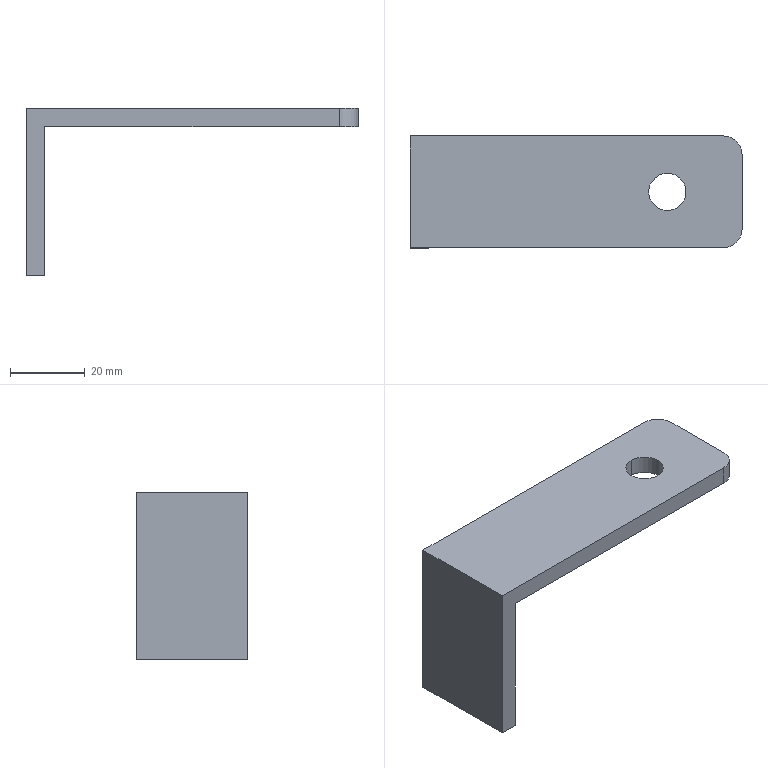Component | SolidWorks | PullPlate-1 | 1 solid | 12 faces | box 89 x 30 x 45 mm | volume 18904 mm3 | plane 8 | cylinder 4 | commonest cylinder face diameters 10 x4 | material 45
build123d program:
from build123d import *

# Parameters (mm, degrees)
BOSS_EXTRUDE1_DEPTH = 30
FILLET1_R           = 5
CUT_EXTRUDE1_REACH  = 101.905
SKETCH2_R           = 5


with BuildPart() as part:
    # Sketch1 → Boss-Extrude1 (new body)
    with BuildSketch(Plane.XY):
        Polygon((0, 0), (40, 0), (40, -84), (45, -84), (45, 5), (0, 5), align=None)
    extrude(amount=BOSS_EXTRUDE1_DEPTH)

    # Fillet1
    fillet1_edges = [part.edges().sort_by_distance(p)[0] for p in [
        (42.5, -84, 30),
        (42.5, -84, 0),
    ]]
    fillet(fillet1_edges, radius=FILLET1_R)

    # Sketch2 → Cut-Extrude1 (cut, up to next)
    with BuildSketch(Plane(origin=(45, 0, 0), x_dir=(0, 0, -1), z_dir=(1, 0, 0)), mode=Mode.PRIVATE) as cut_extrude1_sk1:
        with Locations((-15, -64)):
            Circle(SKETCH2_R)
    cut_extrude1_tool1 = extrude(cut_extrude1_sk1.sketch, amount=-CUT_EXTRUDE1_REACH, mode=Mode.PRIVATE) & part.part
    add(cut_extrude1_tool1.solids().sort_by_distance((45, -64, 15))[0], mode=Mode.SUBTRACT)


solid = part.part

# Placed as in the assembly
solid = solid.moved(Location((-228.359, -52.285, 1021), (90, 0, 90)))
STEP:
#1=COLOUR_RGB('',0.7922,0.8196,0.9333);
#2=FILL_AREA_STYLE_COLOUR('',#1);
#3=FILL_AREA_STYLE('',(#2));
#4=SURFACE_STYLE_FILL_AREA(#3);
#5=SURFACE_SIDE_STYLE('',(#4));
#6=SURFACE_STYLE_USAGE(.BOTH.,#5);
#7=PRESENTATION_STYLE_ASSIGNMENT((#6));
#8=CARTESIAN_POINT('',(-6.471,-2.452,41.772));
#9=VERTEX_POINT('',#8);
#10=CARTESIAN_POINT('',(-6.471,-2.846,41.772));
#11=VERTEX_POINT('',#10);
#12=CARTESIAN_POINT('',(-6.471,-2.649,41.772));
#13=DIRECTION('',(0.,-0.,-1.));
#14=DIRECTION('',(-1.,0.,0.));
#15=AXIS2_PLACEMENT_3D('',#12,#13,#14);
#16=CIRCLE('',#15,0.1969);
#17=EDGE_CURVE('',#9,#11,#16,.T.);
#18=ORIENTED_EDGE('',*,*,#17,.T.);
#19=CARTESIAN_POINT('',(-6.471,-2.846,41.969));
#20=VERTEX_POINT('',#19);
#21=CARTESIAN_POINT('',(-6.471,-2.846,40.197));
#22=DIRECTION('',(0.,0.,1.));
#23=VECTOR('',#22,39.37);
#24=LINE('',#21,#23);
#25=EDGE_CURVE('',#11,#20,#24,.T.);
#26=ORIENTED_EDGE('',*,*,#25,.T.);
#27=CARTESIAN_POINT('',(-6.471,-2.452,41.969));
#28=VERTEX_POINT('',#27);
#29=CARTESIAN_POINT('',(-6.471,-2.649,41.969));
#30=DIRECTION('',(0.,0.,1.));
#31=DIRECTION('',(0.,1.,0.));
#32=AXIS2_PLACEMENT_3D('',#29,#30,#31);
#33=CIRCLE('',#32,0.1969);
#34=EDGE_CURVE('',#20,#28,#33,.T.);
#35=ORIENTED_EDGE('',*,*,#34,.T.);
#36=CARTESIAN_POINT('',(-6.471,-2.452,40.197));
#37=DIRECTION('',(0.,0.,1.));
#38=VECTOR('',#37,39.37);
#39=LINE('',#36,#38);
#40=EDGE_CURVE('',#9,#28,#39,.T.);
#41=ORIENTED_EDGE('',*,*,#40,.F.);
#42=EDGE_LOOP('',(#18,#26,#35,#41));
#43=FACE_OUTER_BOUND('',#42,.T.);
#44=CARTESIAN_POINT('',(-6.471,-2.649,40.197));
#45=DIRECTION('',(0.,0.,1.));
#46=DIRECTION('',(0.,1.,0.));
#47=AXIS2_PLACEMENT_3D('',#44,#45,#46);
#48=CYLINDRICAL_SURFACE('',#47,0.1969);
#49=ADVANCED_FACE('',(#43),#48,.F.);
#50=CARTESIAN_POINT('',(-9.187,-2.058,40.197));
#51=VERTEX_POINT('',#50);
#52=CARTESIAN_POINT('',(-8.991,-2.058,40.197));
#53=VERTEX_POINT('',#52);
#54=CARTESIAN_POINT('',(-9.187,-2.058,40.197));
#55=DIRECTION('',(1.,-0.,-0.));
#56=VECTOR('',#55,39.37);
#57=LINE('',#54,#56);
#58=EDGE_CURVE('',#51,#53,#57,.T.);
#59=ORIENTED_EDGE('',*,*,#58,.T.);
#60=CARTESIAN_POINT('',(-8.991,-3.24,40.197));
#61=VERTEX_POINT('',#60);
#62=CARTESIAN_POINT('',(-8.991,-3.24,40.197));
#63=DIRECTION('',(0.,1.,-0.));
#64=VECTOR('',#63,39.37);
#65=LINE('',#62,#64);
#66=EDGE_CURVE('',#61,#53,#65,.T.);
#67=ORIENTED_EDGE('',*,*,#66,.F.);
#68=CARTESIAN_POINT('',(-9.187,-3.24,40.197));
#69=VERTEX_POINT('',#68);
#70=CARTESIAN_POINT('',(-9.187,-3.24,40.197));
#71=DIRECTION('',(1.,-0.,-0.));
#72=VECTOR('',#71,39.37);
#73=LINE('',#70,#72);
#74=EDGE_CURVE('',#69,#61,#73,.T.);
#75=ORIENTED_EDGE('',*,*,#74,.F.);
#76=CARTESIAN_POINT('',(-9.187,-3.24,40.197));
#77=DIRECTION('',(0.,1.,-0.));
#78=VECTOR('',#77,39.37);
#79=LINE('',#76,#78);
#80=EDGE_CURVE('',#69,#51,#79,.T.);
#81=ORIENTED_EDGE('',*,*,#80,.T.);
#82=EDGE_LOOP('',(#59,#67,#75,#81));
#83=FACE_OUTER_BOUND('',#82,.T.);
#84=CARTESIAN_POINT('',(-9.187,-3.24,40.197));
#85=DIRECTION('',(0.,0.,1.));
#86=DIRECTION('',(0.,1.,-0.));
#87=AXIS2_PLACEMENT_3D('',#84,#85,#86);
#88=PLANE('',#87);
#89=ADVANCED_FACE('',(#83),#88,.F.);
#90=CARTESIAN_POINT('',(-8.991,-2.058,41.772));
#91=VERTEX_POINT('',#90);
#92=CARTESIAN_POINT('',(-8.991,-2.058,40.197));
#93=DIRECTION('',(0.,0.,1.));
#94=VECTOR('',#93,39.37);
#95=LINE('',#92,#94);
#96=EDGE_CURVE('',#53,#91,#95,.T.);
#97=ORIENTED_EDGE('',*,*,#96,.T.);
#98=CARTESIAN_POINT('',(-8.991,-3.24,41.772));
#99=VERTEX_POINT('',#98);
#100=CARTESIAN_POINT('',(-8.991,-3.24,41.772));
#101=DIRECTION('',(0.,1.,-0.));
#102=VECTOR('',#101,39.37);
#103=LINE('',#100,#102);
#104=EDGE_CURVE('',#99,#91,#103,.T.);
#105=ORIENTED_EDGE('',*,*,#104,.F.);
#106=CARTESIAN_POINT('',(-8.991,-3.24,40.197));
#107=DIRECTION('',(0.,0.,1.));
#108=VECTOR('',#107,39.37);
#109=LINE('',#106,#108);
#110=EDGE_CURVE('',#61,#99,#109,.T.);
#111=ORIENTED_EDGE('',*,*,#110,.F.);
#112=ORIENTED_EDGE('',*,*,#66,.T.);
#113=EDGE_LOOP('',(#97,#105,#111,#112));
#114=FACE_OUTER_BOUND('',#113,.T.);
#115=CARTESIAN_POINT('',(-8.991,-3.24,40.197));
#116=DIRECTION('',(-1.,0.,0.));
#117=DIRECTION('',(-0.,-1.,0.));
#118=AXIS2_PLACEMENT_3D('',#115,#116,#117);
#119=PLANE('',#118);
#120=ADVANCED_FACE('',(#114),#119,.F.);
#121=ORIENTED_EDGE('',*,*,#17,.F.);
#122=CARTESIAN_POINT('',(-6.471,-2.649,41.772));
#123=DIRECTION('',(0.,-0.,-1.));
#124=DIRECTION('',(-1.,0.,0.));
#125=AXIS2_PLACEMENT_3D('',#122,#123,#124);
#126=CIRCLE('',#125,0.1969);
#127=EDGE_CURVE('',#11,#9,#126,.T.);
#128=ORIENTED_EDGE('',*,*,#127,.F.);
#129=EDGE_LOOP('',(#121,#128));
#130=FACE_BOUND('',#129,.T.);
#131=CARTESIAN_POINT('',(-5.88,-2.058,41.772));
#132=VERTEX_POINT('',#131);
#133=CARTESIAN_POINT('',(-8.991,-2.058,41.772));
#134=DIRECTION('',(1.,-0.,0.));
#135=VECTOR('',#134,39.37);
#136=LINE('',#133,#135);
#137=EDGE_CURVE('',#91,#132,#136,.T.);
#138=ORIENTED_EDGE('',*,*,#137,.T.);
#139=CARTESIAN_POINT('',(-5.683,-2.255,41.772));
#140=VERTEX_POINT('',#139);
#141=CARTESIAN_POINT('',(-5.88,-2.255,41.772));
#142=DIRECTION('',(0.,-0.,-1.));
#143=DIRECTION('',(-1.,0.,0.));
#144=AXIS2_PLACEMENT_3D('',#141,#142,#143);
#145=CIRCLE('',#144,0.1969);
#146=EDGE_CURVE('',#132,#140,#145,.T.);
#147=ORIENTED_EDGE('',*,*,#146,.T.);
#148=CARTESIAN_POINT('',(-5.683,-3.043,41.772));
#149=VERTEX_POINT('',#148);
#150=CARTESIAN_POINT('',(-5.683,-3.24,41.772));
#151=DIRECTION('',(0.,1.,-0.));
#152=VECTOR('',#151,39.37);
#153=LINE('',#150,#152);
#154=EDGE_CURVE('',#149,#140,#153,.T.);
#155=ORIENTED_EDGE('',*,*,#154,.F.);
#156=CARTESIAN_POINT('',(-5.88,-3.24,41.772));
#157=VERTEX_POINT('',#156);
#158=CARTESIAN_POINT('',(-5.88,-3.043,41.772));
#159=DIRECTION('',(0.,-0.,-1.));
#160=DIRECTION('',(-1.,0.,0.));
#161=AXIS2_PLACEMENT_3D('',#158,#159,#160);
#162=CIRCLE('',#161,0.1969);
#163=EDGE_CURVE('',#149,#157,#162,.T.);
#164=ORIENTED_EDGE('',*,*,#163,.T.);
#165=CARTESIAN_POINT('',(-8.991,-3.24,41.772));
#166=DIRECTION('',(1.,-0.,0.));
#167=VECTOR('',#166,39.37);
#168=LINE('',#165,#167);
#169=EDGE_CURVE('',#99,#157,#168,.T.);
#170=ORIENTED_EDGE('',*,*,#169,.F.);
#171=ORIENTED_EDGE('',*,*,#104,.T.);
#172=EDGE_LOOP('',(#138,#147,#155,#164,#170,#171));
#173=FACE_OUTER_BOUND('',#172,.T.);
#174=CARTESIAN_POINT('',(-8.991,-3.24,41.772));
#175=DIRECTION('',(-0.,0.,1.));
#176=DIRECTION('',(-1.,0.,-0.));
#177=AXIS2_PLACEMENT_3D('',#174,#175,#176);
#178=PLANE('',#177);
#179=ADVANCED_FACE('',(#130,#173),#178,.F.);
#180=ORIENTED_EDGE('',*,*,#154,.T.);
#181=CARTESIAN_POINT('',(-5.683,-2.255,41.969));
#182=VERTEX_POINT('',#181);
#183=CARTESIAN_POINT('',(-5.683,-2.255,41.772));
#184=DIRECTION('',(0.,0.,1.));
#185=VECTOR('',#184,39.37);
#186=LINE('',#183,#185);
#187=EDGE_CURVE('',#140,#182,#186,.T.);
#188=ORIENTED_EDGE('',*,*,#187,.T.);
#189=CARTESIAN_POINT('',(-5.683,-3.043,41.969));
#190=VERTEX_POINT('',#189);
#191=CARTESIAN_POINT('',(-5.683,-3.24,41.969));
#192=DIRECTION('',(0.,1.,-0.));
#193=VECTOR('',#192,39.37);
#194=LINE('',#191,#193);
#195=EDGE_CURVE('',#190,#182,#194,.T.);
#196=ORIENTED_EDGE('',*,*,#195,.F.);
#197=CARTESIAN_POINT('',(-5.683,-3.043,41.772));
#198=DIRECTION('',(-0.,-0.,-1.));
#199=VECTOR('',#198,39.37);
#200=LINE('',#197,#199);
#201=EDGE_CURVE('',#190,#149,#200,.T.);
#202=ORIENTED_EDGE('',*,*,#201,.T.);
#203=EDGE_LOOP('',(#180,#188,#196,#202));
#204=FACE_OUTER_BOUND('',#203,.T.);
#205=CARTESIAN_POINT('',(-5.683,-3.24,41.772));
#206=DIRECTION('',(-1.,0.,0.));
#207=DIRECTION('',(-0.,-1.,0.));
#208=AXIS2_PLACEMENT_3D('',#205,#206,#207);
#209=PLANE('',#208);
#210=ADVANCED_FACE('',(#204),#209,.F.);
#211=CARTESIAN_POINT('',(-6.471,-2.649,41.969));
#212=DIRECTION('',(0.,0.,1.));
#213=DIRECTION('',(0.,1.,0.));
#214=AXIS2_PLACEMENT_3D('',#211,#212,#213);
#215=CIRCLE('',#214,0.1969);
#216=EDGE_CURVE('',#28,#20,#215,.T.);
#217=ORIENTED_EDGE('',*,*,#216,.F.);
#218=ORIENTED_EDGE('',*,*,#34,.F.);
#219=EDGE_LOOP('',(#217,#218));
#220=FACE_BOUND('',#219,.T.);
#221=ORIENTED_EDGE('',*,*,#195,.T.);
#222=CARTESIAN_POINT('',(-5.88,-2.058,41.969));
#223=VERTEX_POINT('',#222);
#224=CARTESIAN_POINT('',(-5.88,-2.255,41.969));
#225=DIRECTION('',(0.,0.,1.));
#226=DIRECTION('',(0.,-1.,0.));
#227=AXIS2_PLACEMENT_3D('',#224,#225,#226);
#228=CIRCLE('',#227,0.1969);
#229=EDGE_CURVE('',#182,#223,#228,.T.);
#230=ORIENTED_EDGE('',*,*,#229,.T.);
#231=CARTESIAN_POINT('',(-9.187,-2.058,41.969));
#232=VERTEX_POINT('',#231);
#233=CARTESIAN_POINT('',(-5.683,-2.058,41.969));
#234=DIRECTION('',(-1.,0.,0.));
#235=VECTOR('',#234,39.37);
#236=LINE('',#233,#235);
#237=EDGE_CURVE('',#223,#232,#236,.T.);
#238=ORIENTED_EDGE('',*,*,#237,.T.);
#239=CARTESIAN_POINT('',(-9.187,-3.24,41.969));
#240=VERTEX_POINT('',#239);
#241=CARTESIAN_POINT('',(-9.187,-3.24,41.969));
#242=DIRECTION('',(0.,1.,-0.));
#243=VECTOR('',#242,39.37);
#244=LINE('',#241,#243);
#245=EDGE_CURVE('',#240,#232,#244,.T.);
#246=ORIENTED_EDGE('',*,*,#245,.F.);
#247=CARTESIAN_POINT('',(-5.88,-3.24,41.969));
#248=VERTEX_POINT('',#247);
#249=CARTESIAN_POINT('',(-5.683,-3.24,41.969));
#250=DIRECTION('',(-1.,0.,0.));
#251=VECTOR('',#250,39.37);
#252=LINE('',#249,#251);
#253=EDGE_CURVE('',#248,#240,#252,.T.);
#254=ORIENTED_EDGE('',*,*,#253,.F.);
#255=CARTESIAN_POINT('',(-5.88,-3.043,41.969));
#256=DIRECTION('',(0.,0.,1.));
#257=DIRECTION('',(0.,-1.,0.));
#258=AXIS2_PLACEMENT_3D('',#255,#256,#257);
#259=CIRCLE('',#258,0.1969);
#260=EDGE_CURVE('',#248,#190,#259,.T.);
#261=ORIENTED_EDGE('',*,*,#260,.T.);
#262=EDGE_LOOP('',(#221,#230,#238,#246,#254,#261));
#263=FACE_OUTER_BOUND('',#262,.T.);
#264=CARTESIAN_POINT('',(-5.683,-3.24,41.969));
#265=DIRECTION('',(-0.,-0.,-1.));
#266=DIRECTION('',(-0.,-1.,0.));
#267=AXIS2_PLACEMENT_3D('',#264,#265,#266);
#268=PLANE('',#267);
#269=ADVANCED_FACE('',(#220,#263),#268,.F.);
#270=CARTESIAN_POINT('',(-9.187,-2.058,41.969));
#271=DIRECTION('',(0.,-0.,-1.));
#272=VECTOR('',#271,39.37);
#273=LINE('',#270,#272);
#274=EDGE_CURVE('',#232,#51,#273,.T.);
#275=ORIENTED_EDGE('',*,*,#274,.T.);
#276=ORIENTED_EDGE('',*,*,#80,.F.);
#277=CARTESIAN_POINT('',(-9.187,-3.24,41.969));
#278=DIRECTION('',(0.,-0.,-1.));
#279=VECTOR('',#278,39.37);
#280=LINE('',#277,#279);
#281=EDGE_CURVE('',#240,#69,#280,.T.);
#282=ORIENTED_EDGE('',*,*,#281,.F.);
#283=ORIENTED_EDGE('',*,*,#245,.T.);
#284=EDGE_LOOP('',(#275,#276,#282,#283));
#285=FACE_OUTER_BOUND('',#284,.T.);
#286=CARTESIAN_POINT('',(-9.187,-3.24,41.969));
#287=DIRECTION('',(1.,-0.,0.));
#288=DIRECTION('',(0.,0.,1.));
#289=AXIS2_PLACEMENT_3D('',#286,#287,#288);
#290=PLANE('',#289);
#291=ADVANCED_FACE('',(#285),#290,.F.);
#292=ORIENTED_EDGE('',*,*,#169,.T.);
#293=CARTESIAN_POINT('',(-5.88,-3.24,41.969));
#294=DIRECTION('',(0.,0.,1.));
#295=VECTOR('',#294,39.37);
#296=LINE('',#293,#295);
#297=EDGE_CURVE('',#157,#248,#296,.T.);
#298=ORIENTED_EDGE('',*,*,#297,.T.);
#299=ORIENTED_EDGE('',*,*,#253,.T.);
#300=ORIENTED_EDGE('',*,*,#281,.T.);
#301=ORIENTED_EDGE('',*,*,#74,.T.);
#302=ORIENTED_EDGE('',*,*,#110,.T.);
#303=EDGE_LOOP('',(#292,#298,#299,#300,#301,#302));
#304=FACE_OUTER_BOUND('',#303,.T.);
#305=CARTESIAN_POINT('',(-8.991,-3.24,40.197));
#306=DIRECTION('',(-0.,-1.,0.));
#307=DIRECTION('',(0.,0.,1.));
#308=AXIS2_PLACEMENT_3D('',#305,#306,#307);
#309=PLANE('',#308);
#310=ADVANCED_FACE('',(#304),#309,.T.);
#311=ORIENTED_EDGE('',*,*,#237,.F.);
#312=CARTESIAN_POINT('',(-5.88,-2.058,40.197));
#313=DIRECTION('',(-0.,-0.,-1.));
#314=VECTOR('',#313,39.37);
#315=LINE('',#312,#314);
#316=EDGE_CURVE('',#223,#132,#315,.T.);
#317=ORIENTED_EDGE('',*,*,#316,.T.);
#318=ORIENTED_EDGE('',*,*,#137,.F.);
#319=ORIENTED_EDGE('',*,*,#96,.F.);
#320=ORIENTED_EDGE('',*,*,#58,.F.);
#321=ORIENTED_EDGE('',*,*,#274,.F.);
#322=EDGE_LOOP('',(#311,#317,#318,#319,#320,#321));
#323=FACE_OUTER_BOUND('',#322,.T.);
#324=CARTESIAN_POINT('',(-8.991,-2.058,40.197));
#325=DIRECTION('',(-0.,-1.,0.));
#326=DIRECTION('',(0.,0.,1.));
#327=AXIS2_PLACEMENT_3D('',#324,#325,#326);
#328=PLANE('',#327);
#329=ADVANCED_FACE('',(#323),#328,.F.);
#330=ORIENTED_EDGE('',*,*,#146,.F.);
#331=ORIENTED_EDGE('',*,*,#316,.F.);
#332=ORIENTED_EDGE('',*,*,#229,.F.);
#333=ORIENTED_EDGE('',*,*,#187,.F.);
#334=EDGE_LOOP('',(#330,#331,#332,#333));
#335=FACE_OUTER_BOUND('',#334,.T.);
#336=CARTESIAN_POINT('',(-5.88,-2.255,41.772));
#337=DIRECTION('',(0.,0.,1.));
#338=DIRECTION('',(0.,1.,0.));
#339=AXIS2_PLACEMENT_3D('',#336,#337,#338);
#340=CYLINDRICAL_SURFACE('',#339,0.1969);
#341=ADVANCED_FACE('',(#335),#340,.T.);
#342=ORIENTED_EDGE('',*,*,#163,.F.);
#343=ORIENTED_EDGE('',*,*,#201,.F.);
#344=ORIENTED_EDGE('',*,*,#260,.F.);
#345=ORIENTED_EDGE('',*,*,#297,.F.);
#346=EDGE_LOOP('',(#342,#343,#344,#345));
#347=FACE_OUTER_BOUND('',#346,.T.);
#348=CARTESIAN_POINT('',(-5.88,-3.043,40.197));
#349=DIRECTION('',(-0.,-0.,-1.));
#350=DIRECTION('',(0.,-1.,0.));
#351=AXIS2_PLACEMENT_3D('',#348,#349,#350);
#352=CYLINDRICAL_SURFACE('',#351,0.1969);
#353=ADVANCED_FACE('',(#347),#352,.T.);
#354=ORIENTED_EDGE('',*,*,#25,.F.);
#355=ORIENTED_EDGE('',*,*,#127,.T.);
#356=ORIENTED_EDGE('',*,*,#40,.T.);
#357=ORIENTED_EDGE('',*,*,#216,.T.);
#358=EDGE_LOOP('',(#354,#355,#356,#357));
#359=FACE_OUTER_BOUND('',#358,.T.);
#360=CARTESIAN_POINT('',(-6.471,-2.649,40.197));
#361=DIRECTION('',(0.,0.,1.));
#362=DIRECTION('',(0.,1.,0.));
#363=AXIS2_PLACEMENT_3D('',#360,#361,#362);
#364=CYLINDRICAL_SURFACE('',#363,0.1969);
#365=ADVANCED_FACE('',(#359),#364,.F.);
#366=CLOSED_SHELL('',(#49,#89,#120,#179,#210,#269,#291,#310,#329,#341,#353,#365));
#367=MANIFOLD_SOLID_BREP('',#366);
#368=STYLED_ITEM('',(#7),#367);
#369=(LENGTH_UNIT()NAMED_UNIT(*)SI_UNIT($,.METRE.));
#370=LENGTH_MEASURE_WITH_UNIT(LENGTH_MEASURE(0.0254),#369);
#371=DIMENSIONAL_EXPONENTS(1.,0.,0.,0.,0.,0.,0.);
#372=(CONVERSION_BASED_UNIT('',#370)LENGTH_UNIT()NAMED_UNIT(#371));
#373=UNCERTAINTY_MEASURE_WITH_UNIT(LENGTH_MEASURE(0.00001),#372,'','');
#374=(NAMED_UNIT(*)PLANE_ANGLE_UNIT()SI_UNIT($,.RADIAN.));
#375=(NAMED_UNIT(*)SI_UNIT($,.STERADIAN.)SOLID_ANGLE_UNIT());
#376=(GEOMETRIC_REPRESENTATION_CONTEXT(3)GLOBAL_UNCERTAINTY_ASSIGNED_CONTEXT((#373))GLOBAL_UNIT_ASSIGNED_CONTEXT((#372,#374,#375))REPRESENTATION_CONTEXT('',''));
#377=MECHANICAL_DESIGN_GEOMETRIC_PRESENTATION_REPRESENTATION('',(#368),#376);
#378=CARTESIAN_POINT('',(0.,0.,0.));
#379=DIRECTION('',(0.,0.,1.));
#380=DIRECTION('',(1.,0.,0.));
#381=AXIS2_PLACEMENT_3D('',#378,#379,#380);
#382=(LENGTH_UNIT()NAMED_UNIT(*)SI_UNIT($,.METRE.));
#383=LENGTH_MEASURE_WITH_UNIT(LENGTH_MEASURE(0.0254),#382);
#384=DIMENSIONAL_EXPONENTS(1.,0.,0.,0.,0.,0.,0.);
#385=(CONVERSION_BASED_UNIT('',#383)LENGTH_UNIT()NAMED_UNIT(#384));
#386=UNCERTAINTY_MEASURE_WITH_UNIT(LENGTH_MEASURE(0.00001),#385,'','');
#387=(NAMED_UNIT(*)PLANE_ANGLE_UNIT()SI_UNIT($,.RADIAN.));
#388=(NAMED_UNIT(*)SI_UNIT($,.STERADIAN.)SOLID_ANGLE_UNIT());
#389=(GEOMETRIC_REPRESENTATION_CONTEXT(3)GLOBAL_UNCERTAINTY_ASSIGNED_CONTEXT((#386))GLOBAL_UNIT_ASSIGNED_CONTEXT((#385,#387,#388))REPRESENTATION_CONTEXT('',''));
#390=ADVANCED_BREP_SHAPE_REPRESENTATION('',(#367,#381),#389);
#391=PRESENTATION_LAYER_ASSIGNMENT('','',(#368));